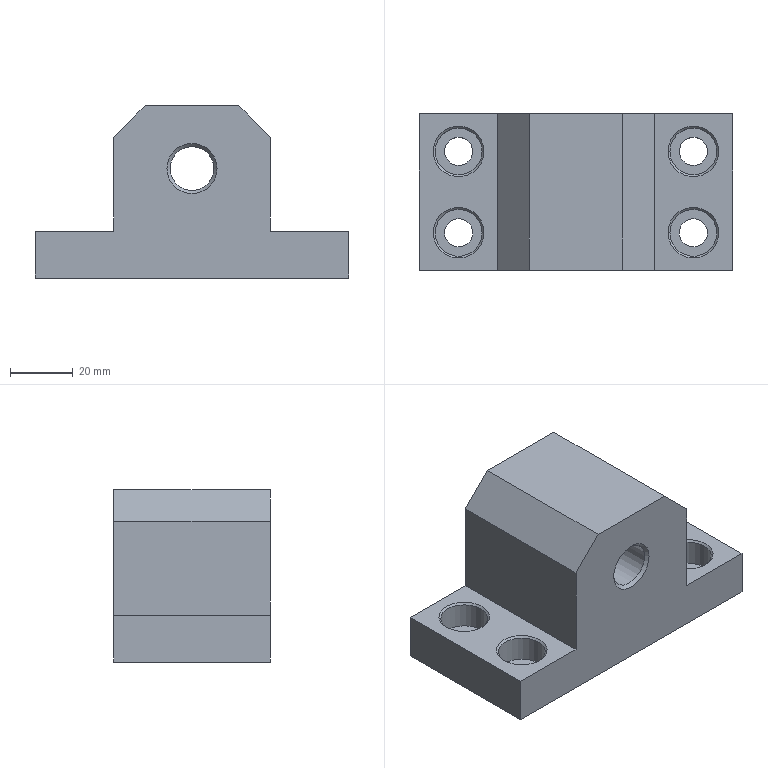Component | NX | FIXED_BRACKET | 1 solid | 35 faces | volume 154403 mm3 | plane 16 | cone 10 | cylinder 9 | commonest cylinder face diameters 9 x4 15 x4 14 x1